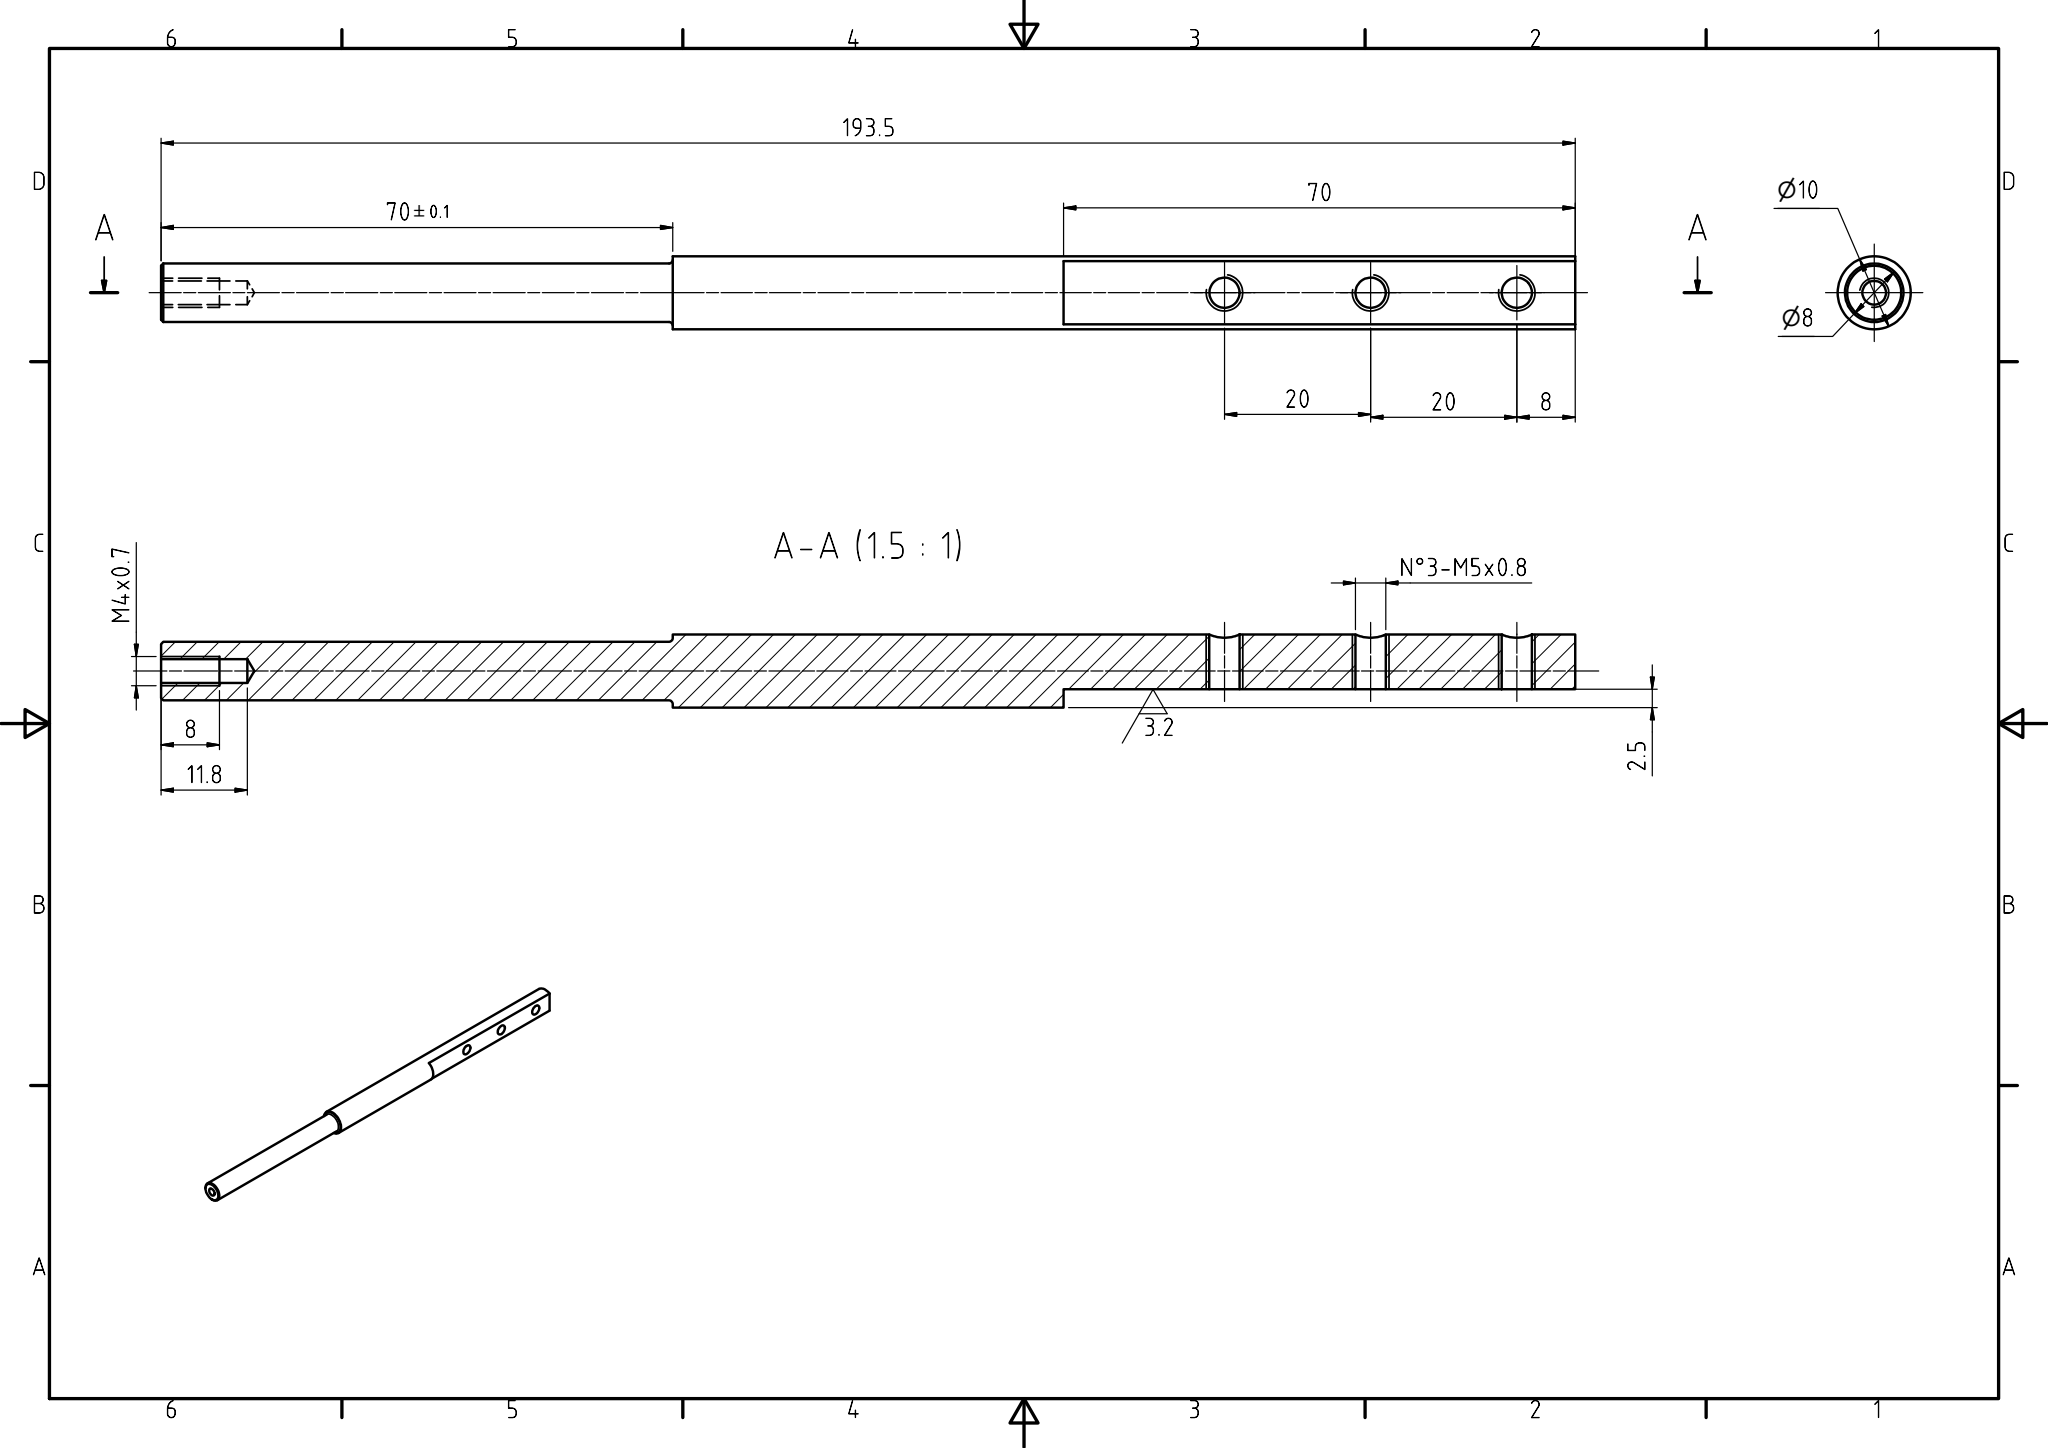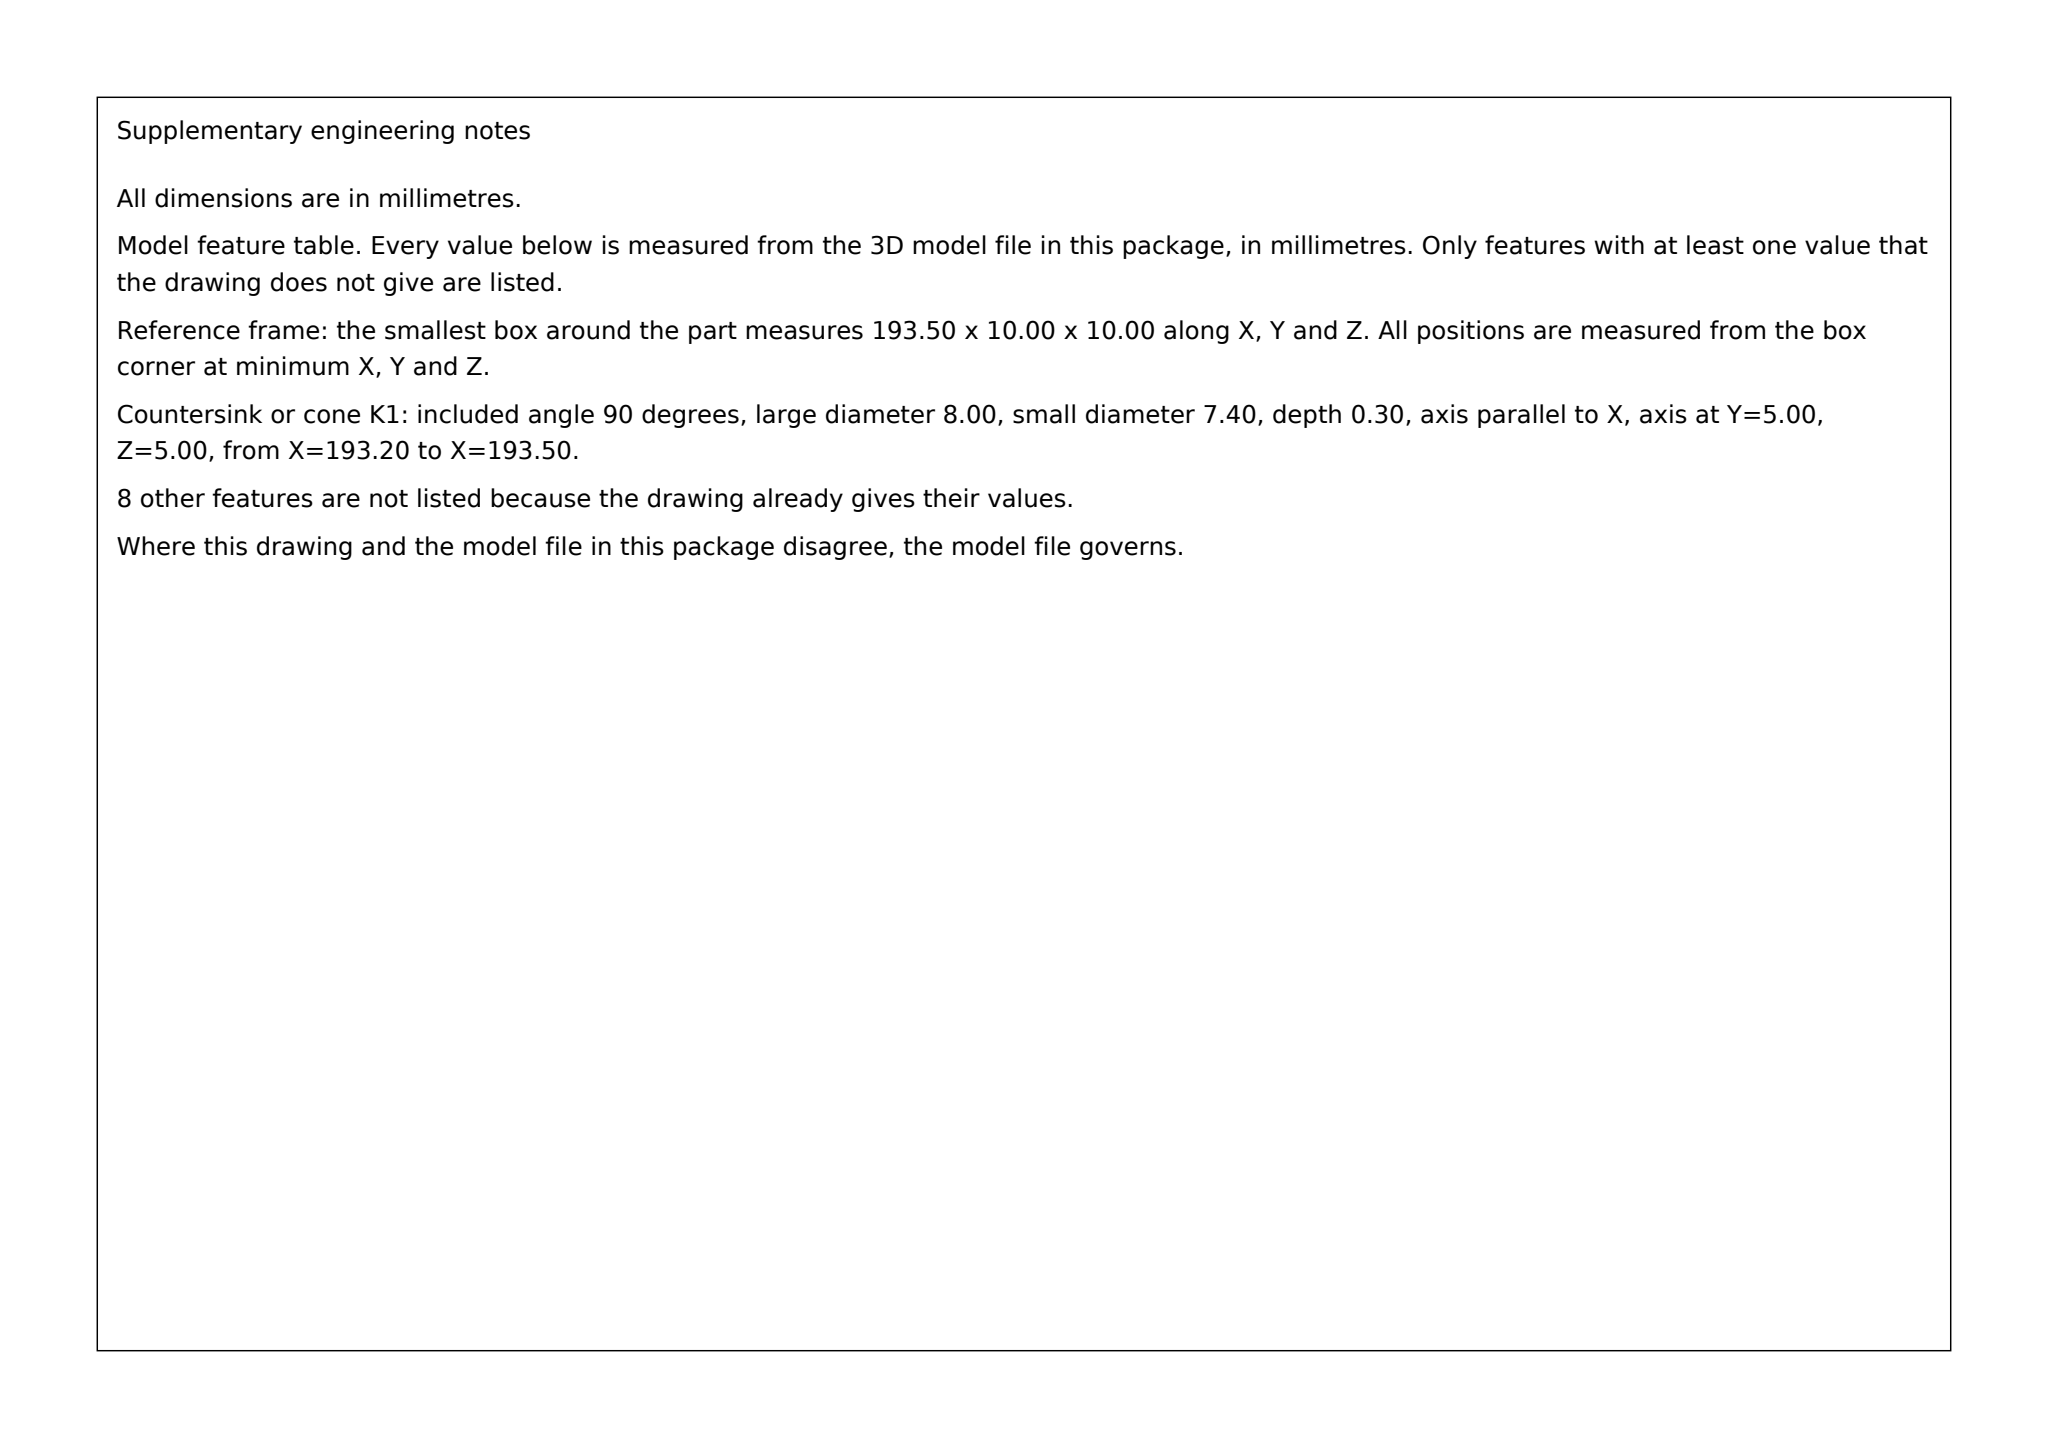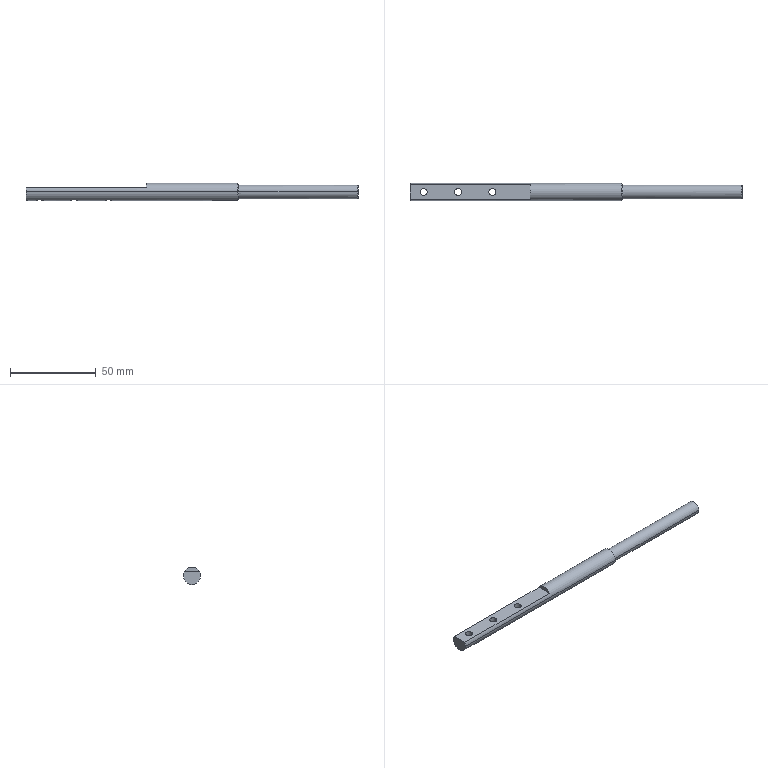Part | SolidWorks | mm | 1 solid | 23 faces | box 193.5 x 10 x 10 mm | volume 11746 mm3 | cylinder 12 | plane 5 | cone 4 | torus 2 | commonest cylinder face diameters 4.134 x6 3.242 x2 10 x2 8 x2